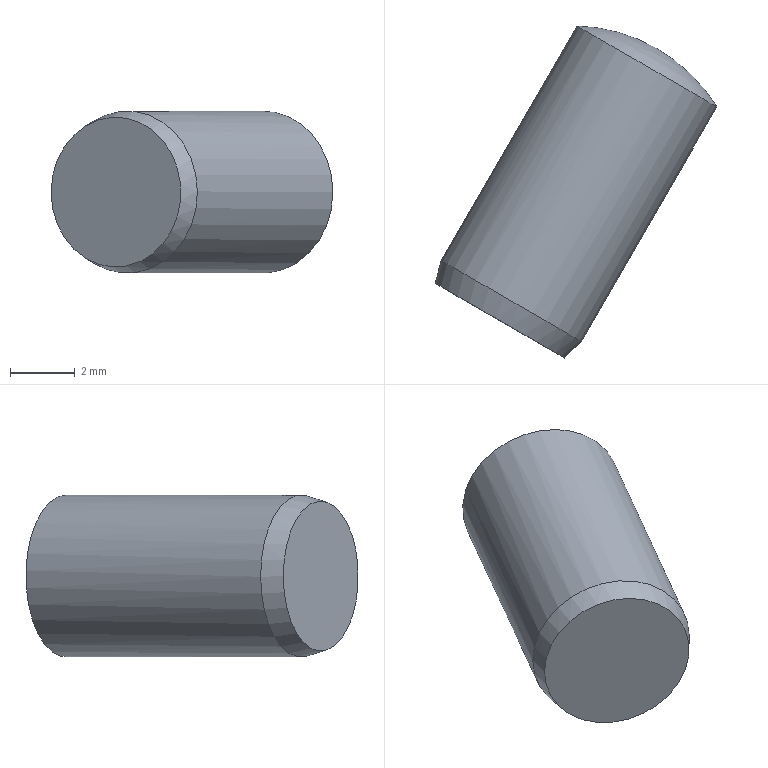Component | NX | CH3404_8-5 | 1 solid | 4 faces | box 8.7 x 10.26 x 5 mm | volume 183 mm3 | sphere 1 | cone 1 | cylinder 1 | plane 1 | commonest cylinder face diameters 5 x1
STEP:
#1=CARTESIAN_POINT('',(0.,0.,0.));
#2=DIRECTION('',(0.,0.,1.));
#3=DIRECTION('',(1.,0.,0.));
#4=AXIS2_PLACEMENT_3D('',#1,#2,#3);
#5=CARTESIAN_POINT('',(19.218,34.365,52.441));
#6=VERTEX_POINT('',#5);
#7=CARTESIAN_POINT('',(21.799,32.875,50.539));
#8=VERTEX_POINT('',#7);
#9=CARTESIAN_POINT('',(19.685,34.095,50.));
#10=DIRECTION('',(-0.5,-0.866,-0.));
#11=DIRECTION('',(0.8456,-0.4882,0.2157));
#12=AXIS2_PLACEMENT_3D('',#9,#10,#11);
#13=CIRCLE('',#12,2.5);
#14=CARTESIAN_POINT('',(17.362,30.072,50.));
#15=DIRECTION('',(-0.5,-0.866,0.));
#16=DIRECTION('',(-0.1868,0.1078,0.9765));
#17=AXIS2_PLACEMENT_3D('',#14,#15,#16);
#18=SPHERICAL_SURFACE('',#17,5.275);
#19=CARTESIAN_POINT('',(-1.571,-1.077));
#20=CARTESIAN_POINT('',(-1.476,-1.077));
#21=CARTESIAN_POINT('',(-1.285,-1.077));
#22=CARTESIAN_POINT('',(-0.9996,-1.077));
#23=CARTESIAN_POINT('',(-0.714,-1.077));
#24=CARTESIAN_POINT('',(-0.4284,-1.077));
#25=CARTESIAN_POINT('',(-0.1428,-1.077));
#26=CARTESIAN_POINT('',(0.1428,-1.077));
#27=CARTESIAN_POINT('',(0.4284,-1.077));
#28=CARTESIAN_POINT('',(0.714,-1.077));
#29=CARTESIAN_POINT('',(0.9996,-1.077));
#30=CARTESIAN_POINT('',(1.285,-1.077));
#31=CARTESIAN_POINT('',(1.571,-1.077));
#32=CARTESIAN_POINT('',(1.856,-1.077));
#33=CARTESIAN_POINT('',(2.142,-1.077));
#34=CARTESIAN_POINT('',(2.428,-1.077));
#35=CARTESIAN_POINT('',(2.713,-1.077));
#36=CARTESIAN_POINT('',(2.999,-1.077));
#37=CARTESIAN_POINT('',(3.284,-1.077));
#38=CARTESIAN_POINT('',(3.57,-1.077));
#39=CARTESIAN_POINT('',(3.856,-1.077));
#40=CARTESIAN_POINT('',(4.141,-1.077));
#41=CARTESIAN_POINT('',(4.427,-1.077));
#42=CARTESIAN_POINT('',(4.617,-1.077));
#43=CARTESIAN_POINT('',(4.712,-1.077));
#44=B_SPLINE_CURVE_WITH_KNOTS('',3,(#19,#20,#21,#22,#23,#24,#25,#26,#27,#28,#29,#30,#31,#32,#33,#34,#35,#36,#37,#38,#39,#40,#41,#42,#43),.UNSPECIFIED.,.F.,.F.,(4,1,1,1,1,1,1,1,1,1,1,1,1,1,1,1,1,1,1,1,1,1,4),(0.,0.2856,0.5712,0.8568,1.142,1.428,1.714,1.999,2.285,2.57,2.856,3.142,3.427,3.713,3.998,4.284,4.57,4.855,5.141,5.426,5.712,5.998,6.283),.QUASI_UNIFORM_KNOTS.);
#45=(GEOMETRIC_REPRESENTATION_CONTEXT(2)PARAMETRIC_REPRESENTATION_CONTEXT()REPRESENTATION_CONTEXT('',''));
#46=DEFINITIONAL_REPRESENTATION('',(#44),#45);
#47=PCURVE('',#18,#46);
#48=CARTESIAN_POINT('',(15.,25.981,50.));
#49=DIRECTION('',(-0.5,-0.866,0.));
#50=DIRECTION('',(0.8456,-0.4882,0.2157));
#51=AXIS2_PLACEMENT_3D('',#48,#49,#50);
#52=CYLINDRICAL_SURFACE('',#51,2.5);
#53=CARTESIAN_POINT('',(0.,-9.37));
#54=DIRECTION('',(1.,0.));
#55=VECTOR('',#54,1.);
#56=LINE('',#53,#55);
#57=(GEOMETRIC_REPRESENTATION_CONTEXT(2)PARAMETRIC_REPRESENTATION_CONTEXT()REPRESENTATION_CONTEXT('',''));
#58=DEFINITIONAL_REPRESENTATION('',(#56),#57);
#59=PCURVE('',#52,#58);
#60=SURFACE_CURVE('',#13,(#47,#59),.PCURVE_S1.);
#61=EDGE_CURVE('',#6,#8,#60,.T.);
#62=ORIENTED_EDGE('',*,*,#61,.F.);
#63=CARTESIAN_POINT('',(20.,34.641,50.));
#64=VERTEX_POINT('',#63);
#65=CARTESIAN_POINT('',(20.,34.641,50.));
#66=CARTESIAN_POINT('',(19.903,34.697,50.509));
#67=CARTESIAN_POINT('',(19.773,34.698,51.017));
#68=CARTESIAN_POINT('',(19.614,34.641,51.516));
#69=CARTESIAN_POINT('',(19.427,34.529,51.993));
#70=CARTESIAN_POINT('',(19.218,34.365,52.441));
#71=B_SPLINE_CURVE_WITH_KNOTS('',5,(#65,#66,#67,#68,#69,#70),.UNSPECIFIED.,.F.,.F.,(6,6),(-1.571,-1.077),.PIECEWISE_BEZIER_KNOTS.);
#72=CARTESIAN_POINT('',(0.,0.));
#73=DIRECTION('',(0.,1.));
#74=VECTOR('',#73,1.);
#75=LINE('',#72,#74);
#76=(GEOMETRIC_REPRESENTATION_CONTEXT(2)PARAMETRIC_REPRESENTATION_CONTEXT()REPRESENTATION_CONTEXT('',''));
#77=DEFINITIONAL_REPRESENTATION('',(#75),#76);
#78=PCURVE('',#18,#77);
#79=CARTESIAN_POINT('',(6.283,0.));
#80=DIRECTION('',(0.,1.));
#81=VECTOR('',#80,1.);
#82=LINE('',#79,#81);
#83=(GEOMETRIC_REPRESENTATION_CONTEXT(2)PARAMETRIC_REPRESENTATION_CONTEXT()REPRESENTATION_CONTEXT('',''));
#84=DEFINITIONAL_REPRESENTATION('',(#82),#83);
#85=PCURVE('',#18,#84);
#86=SEAM_CURVE('',#71,(#78,#85),.PCURVE_S1.);
#87=EDGE_CURVE('',#64,#6,#86,.T.);
#88=ORIENTED_EDGE('',*,*,#87,.F.);
#89=ORIENTED_EDGE('',*,*,#87,.T.);
#90=CARTESIAN_POINT('',(19.685,34.095,50.));
#91=DIRECTION('',(-0.5,-0.866,-0.));
#92=DIRECTION('',(0.8456,-0.4882,0.2157));
#93=AXIS2_PLACEMENT_3D('',#90,#91,#92);
#94=CIRCLE('',#93,2.5);
#95=CARTESIAN_POINT('',(4.712,-1.077));
#96=CARTESIAN_POINT('',(4.808,-1.077));
#97=CARTESIAN_POINT('',(4.998,-1.077));
#98=CARTESIAN_POINT('',(5.284,-1.077));
#99=CARTESIAN_POINT('',(5.569,-1.077));
#100=CARTESIAN_POINT('',(5.855,-1.077));
#101=CARTESIAN_POINT('',(6.14,-1.077));
#102=CARTESIAN_POINT('',(6.426,-1.077));
#103=CARTESIAN_POINT('',(6.712,-1.077));
#104=CARTESIAN_POINT('',(6.997,-1.077));
#105=CARTESIAN_POINT('',(7.283,-1.077));
#106=CARTESIAN_POINT('',(7.568,-1.077));
#107=CARTESIAN_POINT('',(7.854,-1.077));
#108=CARTESIAN_POINT('',(8.14,-1.077));
#109=CARTESIAN_POINT('',(8.425,-1.077));
#110=CARTESIAN_POINT('',(8.711,-1.077));
#111=CARTESIAN_POINT('',(8.996,-1.077));
#112=CARTESIAN_POINT('',(9.282,-1.077));
#113=CARTESIAN_POINT('',(9.568,-1.077));
#114=CARTESIAN_POINT('',(9.853,-1.077));
#115=CARTESIAN_POINT('',(10.139,-1.077));
#116=CARTESIAN_POINT('',(10.424,-1.077));
#117=CARTESIAN_POINT('',(10.71,-1.077));
#118=CARTESIAN_POINT('',(10.9,-1.077));
#119=CARTESIAN_POINT('',(10.996,-1.077));
#120=B_SPLINE_CURVE_WITH_KNOTS('',3,(#95,#96,#97,#98,#99,#100,#101,#102,#103,#104,#105,#106,#107,#108,#109,#110,#111,#112,#113,#114,#115,#116,#117,#118,#119),.UNSPECIFIED.,.F.,.F.,(4,1,1,1,1,1,1,1,1,1,1,1,1,1,1,1,1,1,1,1,1,1,4),(0.,0.2856,0.5712,0.8568,1.142,1.428,1.714,1.999,2.285,2.57,2.856,3.142,3.427,3.713,3.998,4.284,4.57,4.855,5.141,5.426,5.712,5.998,6.283),.QUASI_UNIFORM_KNOTS.);
#121=(GEOMETRIC_REPRESENTATION_CONTEXT(2)PARAMETRIC_REPRESENTATION_CONTEXT()REPRESENTATION_CONTEXT('',''));
#122=DEFINITIONAL_REPRESENTATION('',(#120),#121);
#123=PCURVE('',#18,#122);
#124=CARTESIAN_POINT('',(0.,-9.37));
#125=DIRECTION('',(1.,0.));
#126=VECTOR('',#125,1.);
#127=LINE('',#124,#126);
#128=(GEOMETRIC_REPRESENTATION_CONTEXT(2)PARAMETRIC_REPRESENTATION_CONTEXT()REPRESENTATION_CONTEXT('',''));
#129=DEFINITIONAL_REPRESENTATION('',(#127),#128);
#130=PCURVE('',#52,#129);
#131=SURFACE_CURVE('',#94,(#123,#130),.PCURVE_S1.);
#132=EDGE_CURVE('',#8,#6,#131,.T.);
#133=ORIENTED_EDGE('',*,*,#132,.F.);
#134=EDGE_LOOP('',(#62,#88,#89,#133));
#135=FACE_BOUND('',#134,.T.);
#136=ADVANCED_FACE('',(#135),#18,.T.);
#137=CARTESIAN_POINT('',(13.194,27.37,49.501));
#138=VERTEX_POINT('',#137);
#139=CARTESIAN_POINT('',(15.15,26.241,50.));
#140=DIRECTION('',(-0.5,-0.866,0.));
#141=DIRECTION('',(-0.8456,0.4882,-0.2157));
#142=AXIS2_PLACEMENT_3D('',#139,#140,#141);
#143=CIRCLE('',#142,2.312);
#144=CARTESIAN_POINT('',(15.,25.981,50.));
#145=DIRECTION('',(0.5,0.866,0.));
#146=DIRECTION('',(-0.8456,0.4882,-0.2157));
#147=AXIS2_PLACEMENT_3D('',#144,#145,#146);
#148=CONICAL_SURFACE('',#147,2.232,0.2618);
#149=CARTESIAN_POINT('',(6.283,0.3));
#150=DIRECTION('',(-1.,0.));
#151=VECTOR('',#150,1.);
#152=LINE('',#149,#151);
#153=(GEOMETRIC_REPRESENTATION_CONTEXT(2)PARAMETRIC_REPRESENTATION_CONTEXT()REPRESENTATION_CONTEXT('',''));
#154=DEFINITIONAL_REPRESENTATION('',(#152),#153);
#155=PCURVE('',#148,#154);
#156=CARTESIAN_POINT('',(15.15,26.241,50.));
#157=DIRECTION('',(0.5,0.866,0.));
#158=DIRECTION('',(-0.8456,0.4882,-0.2157));
#159=AXIS2_PLACEMENT_3D('',#156,#157,#158);
#160=PLANE('',#159);
#161=CARTESIAN_POINT('',(2.312,-0.));
#162=CARTESIAN_POINT('',(2.312,-4.005));
#163=CARTESIAN_POINT('',(-1.156,-2.003));
#164=CARTESIAN_POINT('',(-4.625,0.));
#165=CARTESIAN_POINT('',(-1.156,2.003));
#166=CARTESIAN_POINT('',(2.312,4.005));
#167=CARTESIAN_POINT('',(2.312,-0.));
#168=(BOUNDED_CURVE()B_SPLINE_CURVE(2,(#161,#162,#163,#164,#165,#166,#167),.UNSPECIFIED.,.T.,.F.)B_SPLINE_CURVE_WITH_KNOTS((1,2,2,2,2,1),(-2.094,0.,2.094,4.189,6.283,8.378),.UNSPECIFIED.)CURVE()GEOMETRIC_REPRESENTATION_ITEM()RATIONAL_B_SPLINE_CURVE((1.,0.5,1.,0.5,1.,0.5,1.))REPRESENTATION_ITEM(''));
#169=(GEOMETRIC_REPRESENTATION_CONTEXT(2)PARAMETRIC_REPRESENTATION_CONTEXT()REPRESENTATION_CONTEXT('',''));
#170=DEFINITIONAL_REPRESENTATION('',(#168),#169);
#171=PCURVE('',#160,#170);
#172=SURFACE_CURVE('',#143,(#155,#171),.PCURVE_S1.);
#173=EDGE_CURVE('',#138,#138,#172,.T.);
#174=ORIENTED_EDGE('',*,*,#173,.F.);
#175=CARTESIAN_POINT('',(13.386,28.067,49.461));
#176=VERTEX_POINT('',#175);
#177=CARTESIAN_POINT('',(13.194,27.37,49.501));
#178=CARTESIAN_POINT('',(13.386,28.067,49.461));
#179=B_SPLINE_CURVE_WITH_KNOTS('',1,(#177,#178),.UNSPECIFIED.,.F.,.F.,(2,2),(0.3106,1.035),.PIECEWISE_BEZIER_KNOTS.);
#180=CARTESIAN_POINT('',(6.283,0.));
#181=DIRECTION('',(0.,1.));
#182=VECTOR('',#181,1.);
#183=LINE('',#180,#182);
#184=(GEOMETRIC_REPRESENTATION_CONTEXT(2)PARAMETRIC_REPRESENTATION_CONTEXT()REPRESENTATION_CONTEXT('',''));
#185=DEFINITIONAL_REPRESENTATION('',(#183),#184);
#186=PCURVE('',#148,#185);
#187=CARTESIAN_POINT('',(0.,0.));
#188=DIRECTION('',(0.,1.));
#189=VECTOR('',#188,1.);
#190=LINE('',#187,#189);
#191=(GEOMETRIC_REPRESENTATION_CONTEXT(2)PARAMETRIC_REPRESENTATION_CONTEXT()REPRESENTATION_CONTEXT('',''));
#192=DEFINITIONAL_REPRESENTATION('',(#190),#191);
#193=PCURVE('',#148,#192);
#194=SEAM_CURVE('',#179,(#186,#193),.PCURVE_S1.);
#195=EDGE_CURVE('',#138,#176,#194,.T.);
#196=ORIENTED_EDGE('',*,*,#195,.T.);
#197=CARTESIAN_POINT('',(17.614,25.626,50.539));
#198=VERTEX_POINT('',#197);
#199=CARTESIAN_POINT('',(15.5,26.847,50.));
#200=DIRECTION('',(-0.5,-0.866,0.));
#201=DIRECTION('',(0.8456,-0.4882,0.2157));
#202=AXIS2_PLACEMENT_3D('',#199,#200,#201);
#203=CIRCLE('',#202,2.5);
#204=CARTESIAN_POINT('',(9.425,1.));
#205=DIRECTION('',(-1.,0.));
#206=VECTOR('',#205,1.);
#207=LINE('',#204,#206);
#208=(GEOMETRIC_REPRESENTATION_CONTEXT(2)PARAMETRIC_REPRESENTATION_CONTEXT()REPRESENTATION_CONTEXT('',''));
#209=DEFINITIONAL_REPRESENTATION('',(#207),#208);
#210=PCURVE('',#148,#209);
#211=CARTESIAN_POINT('',(0.,-1.));
#212=DIRECTION('',(1.,0.));
#213=VECTOR('',#212,1.);
#214=LINE('',#211,#213);
#215=(GEOMETRIC_REPRESENTATION_CONTEXT(2)PARAMETRIC_REPRESENTATION_CONTEXT()REPRESENTATION_CONTEXT('',''));
#216=DEFINITIONAL_REPRESENTATION('',(#214),#215);
#217=PCURVE('',#52,#216);
#218=SURFACE_CURVE('',#203,(#210,#217),.PCURVE_S1.);
#219=EDGE_CURVE('',#176,#198,#218,.T.);
#220=ORIENTED_EDGE('',*,*,#219,.T.);
#221=CARTESIAN_POINT('',(15.5,26.847,50.));
#222=DIRECTION('',(-0.5,-0.866,0.));
#223=DIRECTION('',(0.8456,-0.4882,0.2157));
#224=AXIS2_PLACEMENT_3D('',#221,#222,#223);
#225=CIRCLE('',#224,2.5);
#226=CARTESIAN_POINT('',(3.142,1.));
#227=DIRECTION('',(-1.,0.));
#228=VECTOR('',#227,1.);
#229=LINE('',#226,#228);
#230=(GEOMETRIC_REPRESENTATION_CONTEXT(2)PARAMETRIC_REPRESENTATION_CONTEXT()REPRESENTATION_CONTEXT('',''));
#231=DEFINITIONAL_REPRESENTATION('',(#229),#230);
#232=PCURVE('',#148,#231);
#233=CARTESIAN_POINT('',(0.,-1.));
#234=DIRECTION('',(1.,0.));
#235=VECTOR('',#234,1.);
#236=LINE('',#233,#235);
#237=(GEOMETRIC_REPRESENTATION_CONTEXT(2)PARAMETRIC_REPRESENTATION_CONTEXT()REPRESENTATION_CONTEXT('',''));
#238=DEFINITIONAL_REPRESENTATION('',(#236),#237);
#239=PCURVE('',#52,#238);
#240=SURFACE_CURVE('',#225,(#232,#239),.PCURVE_S1.);
#241=EDGE_CURVE('',#198,#176,#240,.T.);
#242=ORIENTED_EDGE('',*,*,#241,.T.);
#243=ORIENTED_EDGE('',*,*,#195,.F.);
#244=EDGE_LOOP('',(#174,#196,#220,#242,#243));
#245=FACE_BOUND('',#244,.T.);
#246=ADVANCED_FACE('',(#245),#148,.T.);
#247=ORIENTED_EDGE('',*,*,#132,.T.);
#248=ORIENTED_EDGE('',*,*,#61,.T.);
#249=CARTESIAN_POINT('',(21.799,32.875,50.539));
#250=CARTESIAN_POINT('',(17.614,25.626,50.539));
#251=B_SPLINE_CURVE_WITH_KNOTS('',1,(#249,#250),.UNSPECIFIED.,.F.,.F.,(2,2),(-9.37,-1.),.PIECEWISE_BEZIER_KNOTS.);
#252=CARTESIAN_POINT('',(6.283,0.));
#253=DIRECTION('',(0.,1.));
#254=VECTOR('',#253,1.);
#255=LINE('',#252,#254);
#256=(GEOMETRIC_REPRESENTATION_CONTEXT(2)PARAMETRIC_REPRESENTATION_CONTEXT()REPRESENTATION_CONTEXT('',''));
#257=DEFINITIONAL_REPRESENTATION('',(#255),#256);
#258=PCURVE('',#52,#257);
#259=CARTESIAN_POINT('',(0.,0.));
#260=DIRECTION('',(0.,1.));
#261=VECTOR('',#260,1.);
#262=LINE('',#259,#261);
#263=(GEOMETRIC_REPRESENTATION_CONTEXT(2)PARAMETRIC_REPRESENTATION_CONTEXT()REPRESENTATION_CONTEXT('',''));
#264=DEFINITIONAL_REPRESENTATION('',(#262),#263);
#265=PCURVE('',#52,#264);
#266=SEAM_CURVE('',#251,(#258,#265),.PCURVE_S1.);
#267=EDGE_CURVE('',#8,#198,#266,.T.);
#268=ORIENTED_EDGE('',*,*,#267,.T.);
#269=ORIENTED_EDGE('',*,*,#219,.F.);
#270=ORIENTED_EDGE('',*,*,#241,.F.);
#271=ORIENTED_EDGE('',*,*,#267,.F.);
#272=EDGE_LOOP('',(#247,#248,#268,#269,#270,#271));
#273=FACE_BOUND('',#272,.T.);
#274=ADVANCED_FACE('',(#273),#52,.T.);
#275=ORIENTED_EDGE('',*,*,#173,.T.);
#276=EDGE_LOOP('',(#275));
#277=FACE_BOUND('',#276,.T.);
#278=ADVANCED_FACE('',(#277),#160,.F.);
#279=CLOSED_SHELL('',(#136,#246,#274,#278));
#280=MANIFOLD_SOLID_BREP('',#279);
#281=(LENGTH_UNIT()NAMED_UNIT(*)SI_UNIT(.MILLI.,.METRE.));
#282=UNCERTAINTY_MEASURE_WITH_UNIT(LENGTH_MEASURE(0.00001),#281,'','');
#283=(NAMED_UNIT(*)PLANE_ANGLE_UNIT()SI_UNIT($,.RADIAN.));
#284=(NAMED_UNIT(*)SI_UNIT($,.STERADIAN.)SOLID_ANGLE_UNIT());
#285=(GEOMETRIC_REPRESENTATION_CONTEXT(3)GLOBAL_UNCERTAINTY_ASSIGNED_CONTEXT((#282))GLOBAL_UNIT_ASSIGNED_CONTEXT((#281,#283,#284))REPRESENTATION_CONTEXT('',''));
#286=ADVANCED_BREP_SHAPE_REPRESENTATION('',(#4,#280),#285);